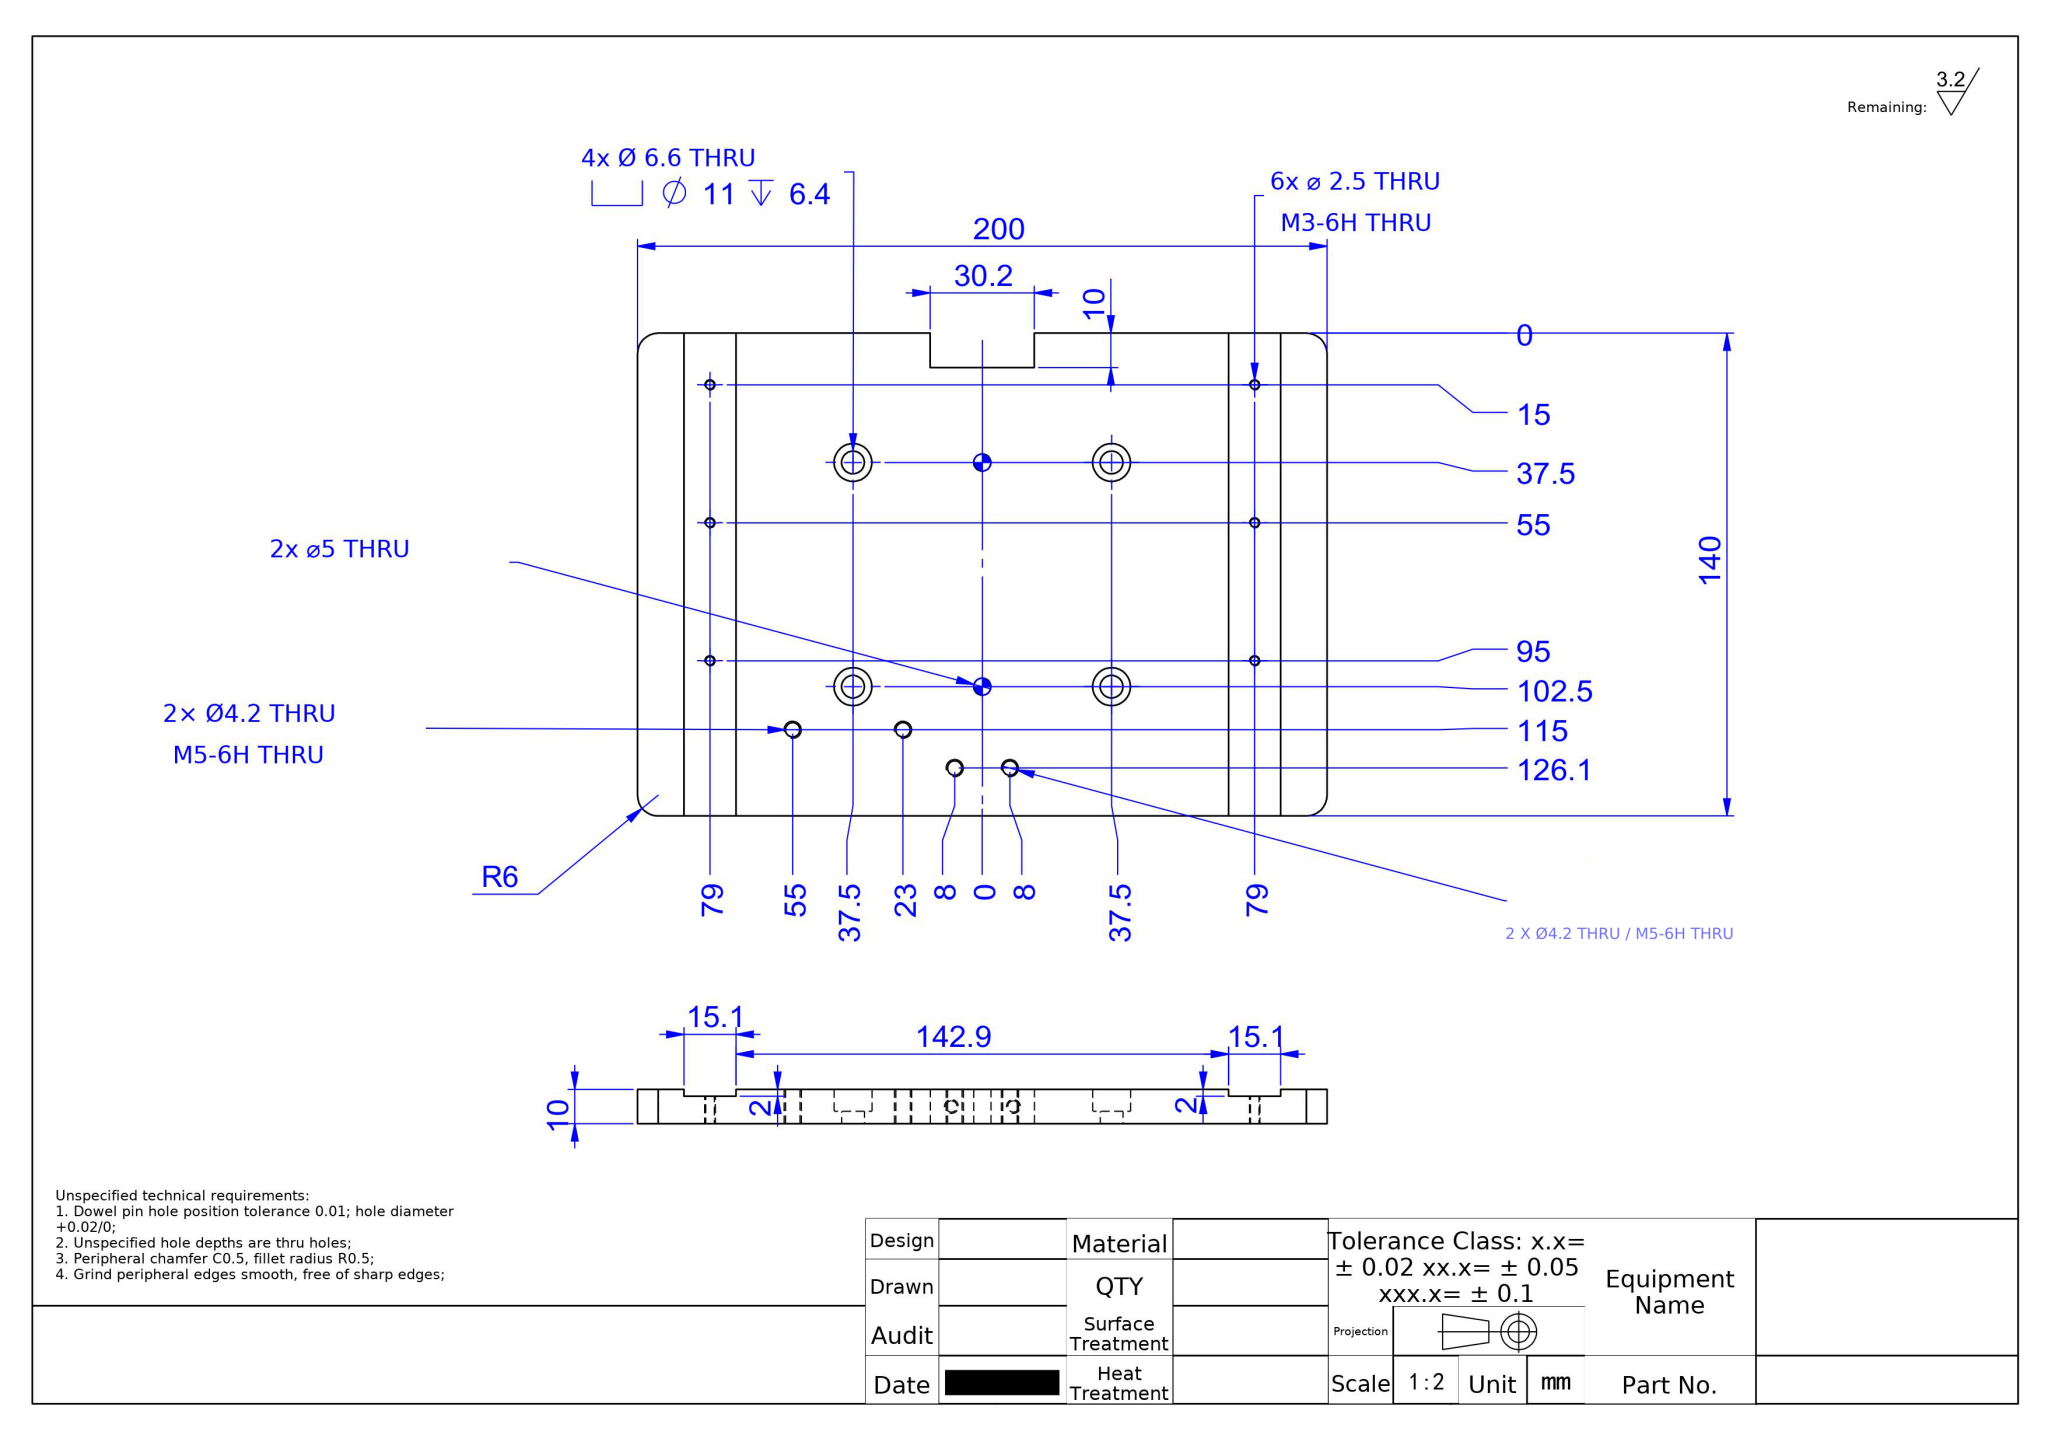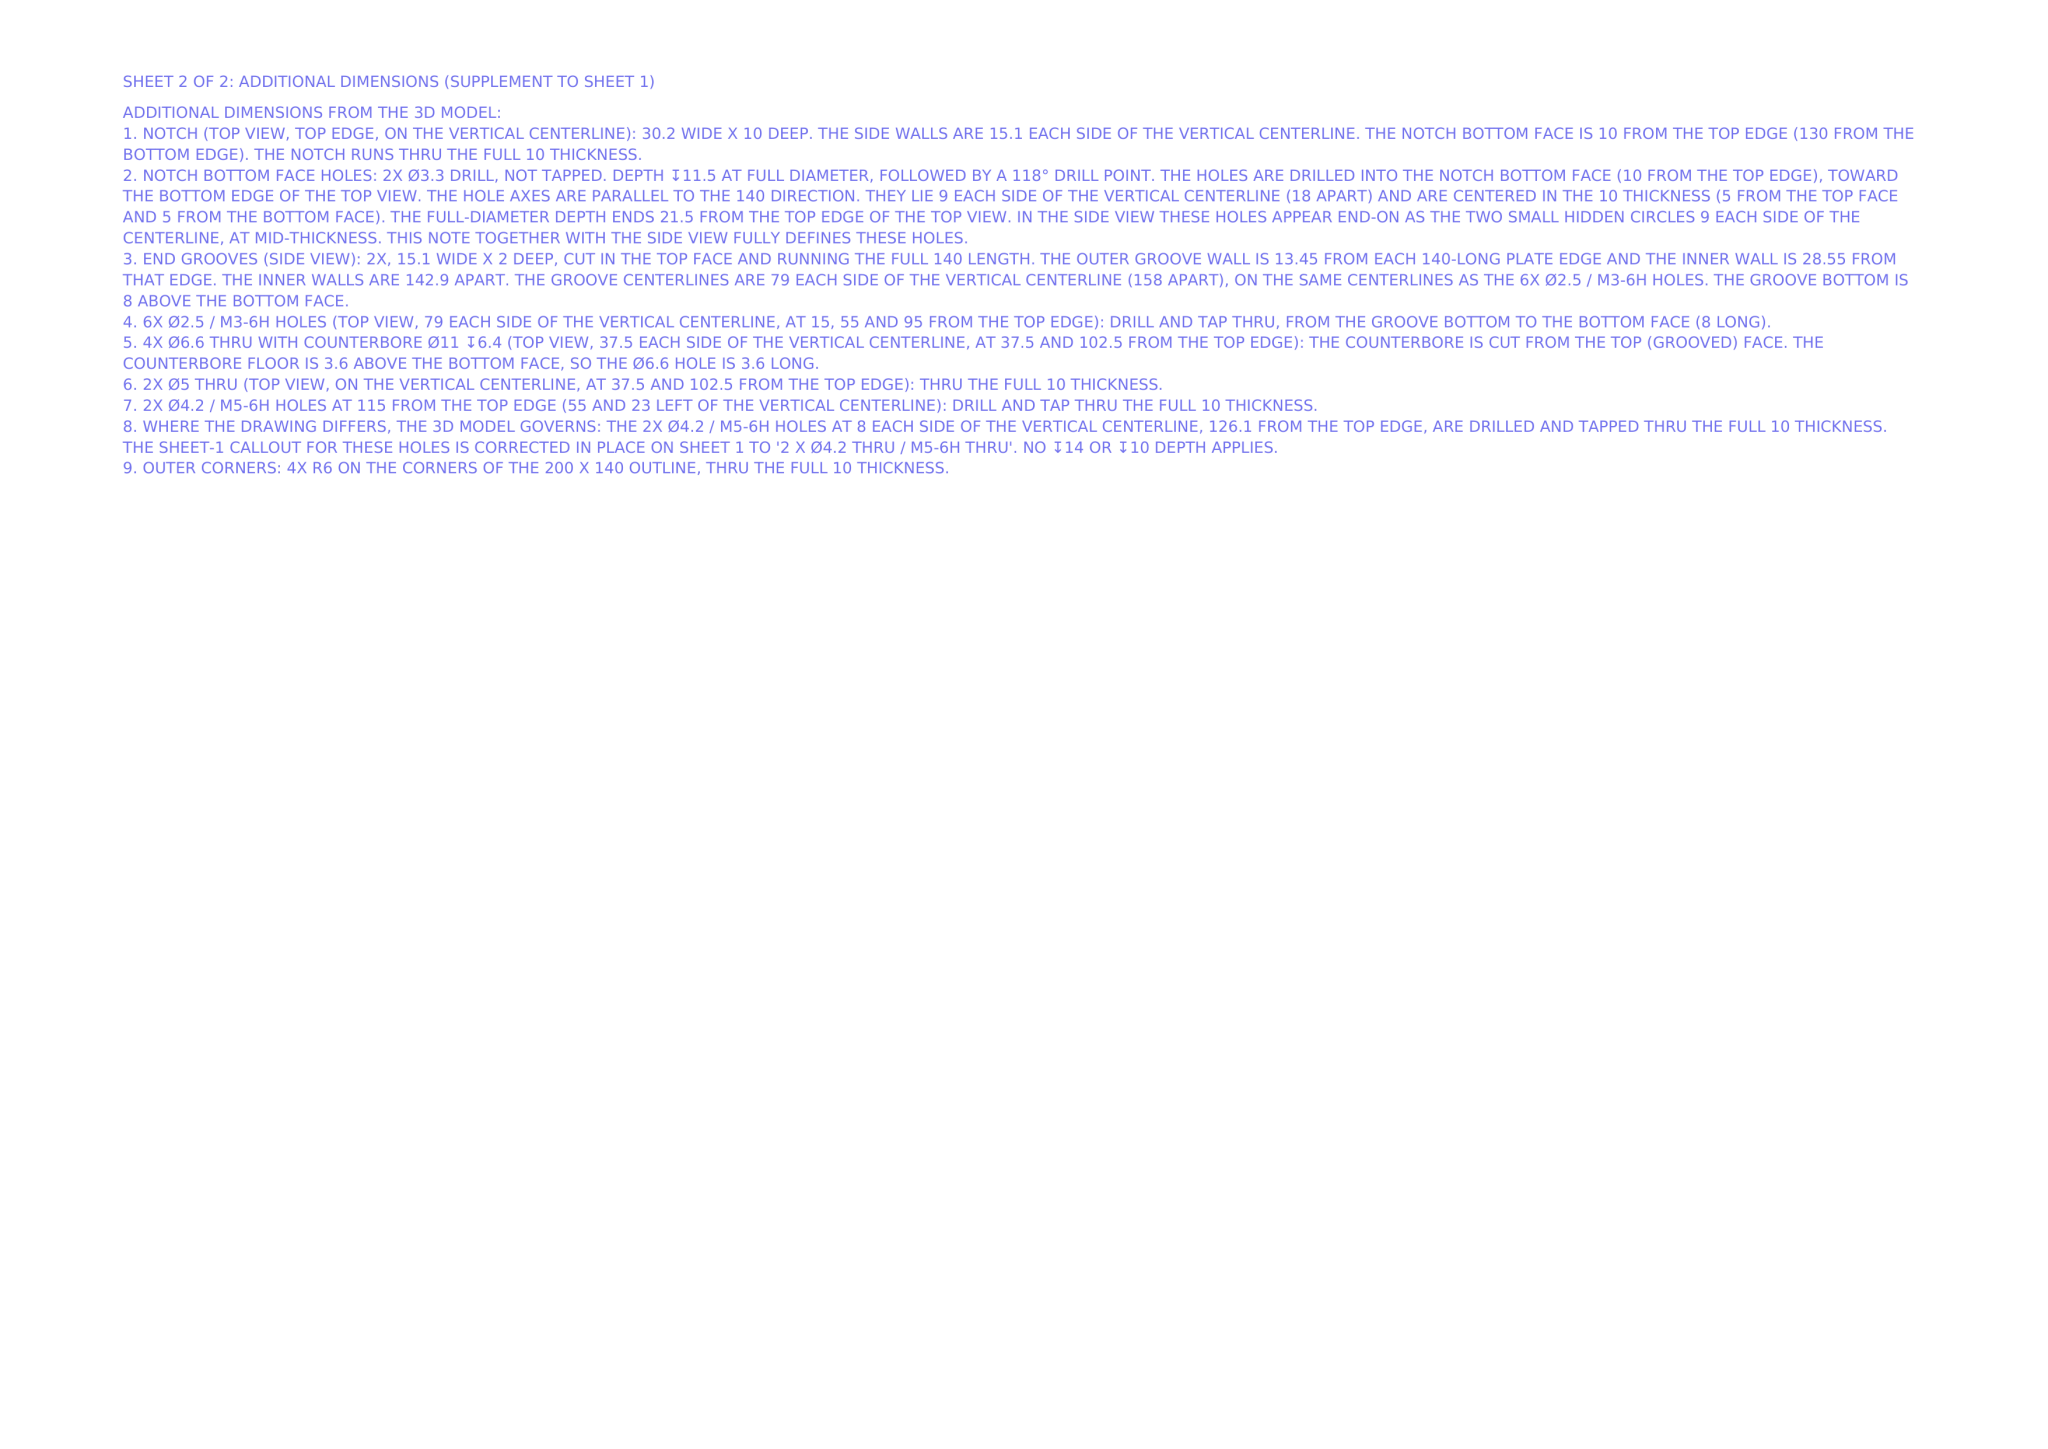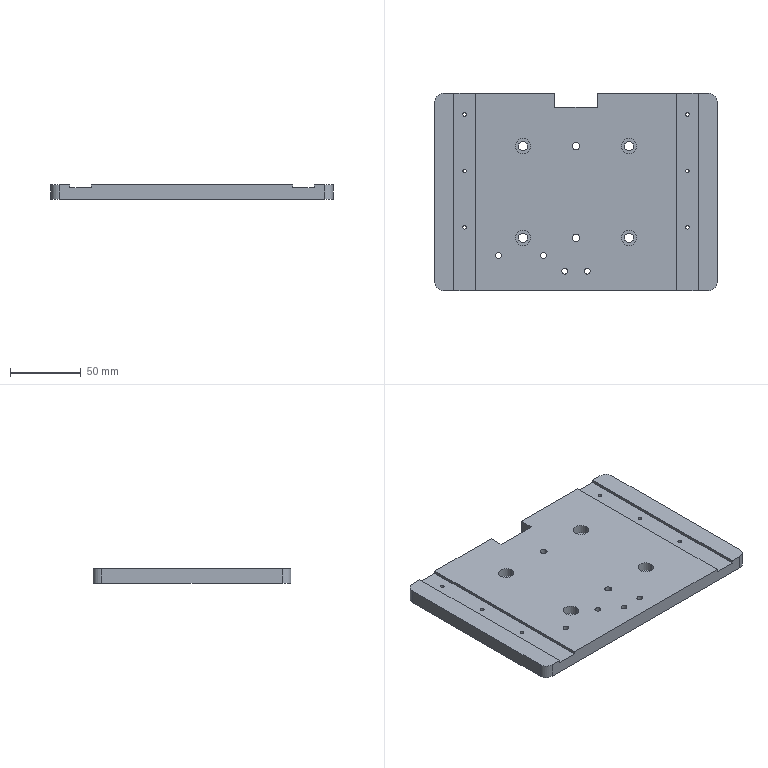Part | NX | mm | 1 solid | 74 faces | box 200 x 140 x 10 mm | volume 263905 mm3 | cylinder 48 | plane 22 | cone 4 | commonest cylinder face diameters 2.5 x12 4.2 x8 11 x8 6.6 x8 3.3 x4 5 x4 12 x4